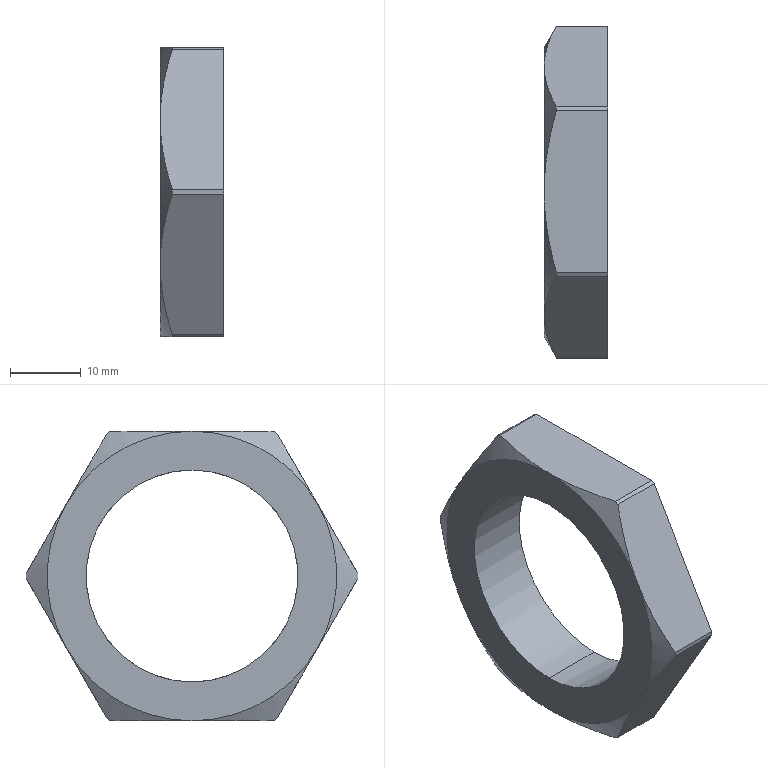Component | SolidWorks | MAL40_M30x2_Nut-1 | 1 solid | 22 faces | box 9 x 47 x 41 mm | volume 6663 mm3 | cylinder 8 | plane 8 | cone 6 | commonest cylinder face diameters 47 x6 30 x2
build123d program:
from build123d import *

# Parameters (mm, degrees)
SKETCH2_W                         = 82
SKETCH2_H                         = 82
EXTRUDE1_DEPTH                    = 18
THREADMAJORDIABORE_M30_DEPTH      = 33.458
THREADMAJORDIABORE_M30_DEPTH_BACK = 33.458
SKETCH4_R                         = 15


with BuildPart() as part:
    # Sketch1 → Revolve1 (revolve)
    with BuildSketch(Plane.XY, mode=Mode.PRIVATE) as revolve1_sk:
        Polygon((0, 0), (0, 20.5), (1.732, 23.5), (9, 23.5), (9, 0), align=None)
    revolve(revolve1_sk.sketch.rotate(Axis((9, 0, 0), (-1, 0, 0)), 270), axis=Axis((9, 0, 0), (-1, 0, 0)))

    # Sketch2 → Extrude1 (cut)
    with BuildSketch(Plane(origin=(0, 0, 0), x_dir=(0, 0, -1), z_dir=(1, 0, 0))):
        Rectangle(SKETCH2_W, SKETCH2_H)
        Polygon((-20.5, 11.836), (-20.5, -11.836), (0, -23.671), (20.5, -11.836), (20.5, 11.836), (0, 23.671), align=None, mode=Mode.SUBTRACT)
    extrude(amount=EXTRUDE1_DEPTH, mode=Mode.SUBTRACT)

    # Sketch3 → Cut-Revolve1 (revolve, cut)
    with BuildSketch(Plane.XY, mode=Mode.PRIVATE) as cut_revolve1_sk:
        Polygon((0, 0), (0, 15), (1.083, 13.918), (7.918, 13.918), (9, 15), (9, 0), align=None)
    revolve(cut_revolve1_sk.sketch.rotate(Axis((9, 0, 0), (-1, 0, 0)), 270), axis=Axis((9, 0, 0), (-1, 0, 0)), mode=Mode.SUBTRACT)

    # Sketch4 → ThreadMajorDiaBore_M30 (cut, two sides: drawn at the far end of the back side and taken through both)
    with BuildSketch(Plane(origin=(0, 0, 0), x_dir=(0, 0, -1), z_dir=(1, 0, 0)).offset(-THREADMAJORDIABORE_M30_DEPTH_BACK)):
        Circle(SKETCH4_R)
    extrude(amount=THREADMAJORDIABORE_M30_DEPTH + THREADMAJORDIABORE_M30_DEPTH_BACK, mode=Mode.SUBTRACT)


solid = part.part

# Placed as in the assembly
solid = solid.moved(Location((-14, 0, 0), (0, 0, 0)))
STEP:
#1=COLOUR_RGB('',0.7922,0.8196,0.9333);
#2=FILL_AREA_STYLE_COLOUR('',#1);
#3=FILL_AREA_STYLE('',(#2));
#4=SURFACE_STYLE_FILL_AREA(#3);
#5=SURFACE_SIDE_STYLE('',(#4));
#6=SURFACE_STYLE_USAGE(.BOTH.,#5);
#7=PRESENTATION_STYLE_ASSIGNMENT((#6));
#8=CARTESIAN_POINT('',(-0.5512,0.,0.5906));
#9=VERTEX_POINT('',#8);
#10=CARTESIAN_POINT('',(-0.5512,0.,-0.5906));
#11=VERTEX_POINT('',#10);
#12=CARTESIAN_POINT('',(-0.5512,0.,0.5906));
#13=CARTESIAN_POINT('',(-0.5512,-0.03877,0.5906));
#14=CARTESIAN_POINT('',(-0.5512,-0.07719,0.5868));
#15=CARTESIAN_POINT('',(-0.5512,-0.1532,0.5716));
#16=CARTESIAN_POINT('',(-0.5512,-0.1902,0.5604));
#17=CARTESIAN_POINT('',(-0.5512,-0.2618,0.5308));
#18=CARTESIAN_POINT('',(-0.5512,-0.2959,0.5126));
#19=CARTESIAN_POINT('',(-0.5512,-0.3603,0.4695));
#20=CARTESIAN_POINT('',(-0.5512,-0.3902,0.445));
#21=CARTESIAN_POINT('',(-0.5512,-0.445,0.3902));
#22=CARTESIAN_POINT('',(-0.5512,-0.4695,0.3603));
#23=CARTESIAN_POINT('',(-0.5512,-0.5126,0.2959));
#24=CARTESIAN_POINT('',(-0.5512,-0.5308,0.2618));
#25=CARTESIAN_POINT('',(-0.5512,-0.5604,0.1902));
#26=CARTESIAN_POINT('',(-0.5512,-0.5716,0.1532));
#27=CARTESIAN_POINT('',(-0.5512,-0.5868,0.07719));
#28=CARTESIAN_POINT('',(-0.5512,-0.5905,0.03876));
#29=CARTESIAN_POINT('',(-0.5512,-0.5906,-0.03876));
#30=CARTESIAN_POINT('',(-0.5512,-0.5868,-0.07719));
#31=CARTESIAN_POINT('',(-0.5512,-0.5716,-0.1532));
#32=CARTESIAN_POINT('',(-0.5512,-0.5604,-0.1902));
#33=CARTESIAN_POINT('',(-0.5512,-0.5308,-0.2618));
#34=CARTESIAN_POINT('',(-0.5512,-0.5126,-0.2959));
#35=CARTESIAN_POINT('',(-0.5512,-0.4695,-0.3603));
#36=CARTESIAN_POINT('',(-0.5512,-0.445,-0.3902));
#37=CARTESIAN_POINT('',(-0.5512,-0.3902,-0.445));
#38=CARTESIAN_POINT('',(-0.5512,-0.3603,-0.4695));
#39=CARTESIAN_POINT('',(-0.5512,-0.2959,-0.5126));
#40=CARTESIAN_POINT('',(-0.5512,-0.2618,-0.5308));
#41=CARTESIAN_POINT('',(-0.5512,-0.1902,-0.5604));
#42=CARTESIAN_POINT('',(-0.5512,-0.1532,-0.5716));
#43=CARTESIAN_POINT('',(-0.5512,-0.07719,-0.5868));
#44=CARTESIAN_POINT('',(-0.5512,-0.03876,-0.5905));
#45=CARTESIAN_POINT('',(-0.5512,0.,-0.5906));
#46=B_SPLINE_CURVE_WITH_KNOTS('',3,(#12,#13,#14,#15,#16,#17,#18,#19,#20,#21,#22,#23,#24,#25,#26,#27,#28,#29,#30,#31,#32,#33,#34,#35,#36,#37,#38,#39,#40,#41,#42,#43,#44,#45),.UNSPECIFIED.,.F.,.F.,(4,2,2,2,2,2,2,2,2,2,2,2,2,2,2,2,4),(0.,0.03125,0.0625,0.09375,0.125,0.1563,0.1875,0.2188,0.25,0.2813,0.3125,0.3438,0.375,0.4063,0.4375,0.4688,0.5),.UNSPECIFIED.);
#47=EDGE_CURVE('',#9,#11,#46,.T.);
#48=ORIENTED_EDGE('',*,*,#47,.F.);
#49=CARTESIAN_POINT('',(-0.1969,0.,0.5906));
#50=VERTEX_POINT('',#49);
#51=CARTESIAN_POINT('',(-0.5512,0.,0.5906));
#52=DIRECTION('',(1.,0.,0.));
#53=VECTOR('',#52,39.37);
#54=LINE('',#51,#53);
#55=EDGE_CURVE('',#9,#50,#54,.T.);
#56=ORIENTED_EDGE('',*,*,#55,.T.);
#57=CARTESIAN_POINT('',(-0.1969,0.,-0.5906));
#58=VERTEX_POINT('',#57);
#59=CARTESIAN_POINT('',(-0.1969,0.,0.));
#60=DIRECTION('',(1.,0.,0.));
#61=DIRECTION('',(0.,0.,-1.));
#62=AXIS2_PLACEMENT_3D('',#59,#60,#61);
#63=CIRCLE('',#62,0.5906);
#64=EDGE_CURVE('',#50,#58,#63,.T.);
#65=ORIENTED_EDGE('',*,*,#64,.T.);
#66=CARTESIAN_POINT('',(-0.5512,0.,-0.5906));
#67=DIRECTION('',(1.,0.,0.));
#68=VECTOR('',#67,39.37);
#69=LINE('',#66,#68);
#70=EDGE_CURVE('',#11,#58,#69,.T.);
#71=ORIENTED_EDGE('',*,*,#70,.F.);
#72=EDGE_LOOP('',(#48,#56,#65,#71));
#73=FACE_OUTER_BOUND('',#72,.T.);
#74=CARTESIAN_POINT('',(-0.5512,0.,0.));
#75=DIRECTION('',(1.,0.,0.));
#76=DIRECTION('',(0.,0.,-1.));
#77=AXIS2_PLACEMENT_3D('',#74,#75,#76);
#78=CYLINDRICAL_SURFACE('',#77,0.5906);
#79=ADVANCED_FACE('',(#73),#78,.F.);
#80=CARTESIAN_POINT('',(-0.5512,0.,0.8071));
#81=VERTEX_POINT('',#80);
#82=CARTESIAN_POINT('',(-0.5512,0.699,0.4035));
#83=VERTEX_POINT('',#82);
#84=CARTESIAN_POINT('',(-0.5512,0.,0.));
#85=DIRECTION('',(-1.,0.,0.));
#86=DIRECTION('',(0.,0.,1.));
#87=AXIS2_PLACEMENT_3D('',#84,#85,#86);
#88=CIRCLE('',#87,0.8071);
#89=EDGE_CURVE('',#81,#83,#88,.T.);
#90=ORIENTED_EDGE('',*,*,#89,.T.);
#91=CARTESIAN_POINT('',(-0.5512,0.699,-0.4035));
#92=VERTEX_POINT('',#91);
#93=CARTESIAN_POINT('',(-0.5512,0.,0.));
#94=DIRECTION('',(-1.,0.,0.));
#95=DIRECTION('',(0.,0.,1.));
#96=AXIS2_PLACEMENT_3D('',#93,#94,#95);
#97=CIRCLE('',#96,0.8071);
#98=EDGE_CURVE('',#83,#92,#97,.T.);
#99=ORIENTED_EDGE('',*,*,#98,.T.);
#100=CARTESIAN_POINT('',(-0.5512,0.,-0.8071));
#101=VERTEX_POINT('',#100);
#102=CARTESIAN_POINT('',(-0.5512,0.,0.));
#103=DIRECTION('',(-1.,0.,0.));
#104=DIRECTION('',(0.,0.,1.));
#105=AXIS2_PLACEMENT_3D('',#102,#103,#104);
#106=CIRCLE('',#105,0.8071);
#107=EDGE_CURVE('',#92,#101,#106,.T.);
#108=ORIENTED_EDGE('',*,*,#107,.T.);
#109=CARTESIAN_POINT('',(-0.5512,-0.699,-0.4035));
#110=VERTEX_POINT('',#109);
#111=CARTESIAN_POINT('',(-0.5512,0.,0.));
#112=DIRECTION('',(-1.,0.,0.));
#113=DIRECTION('',(0.,0.,1.));
#114=AXIS2_PLACEMENT_3D('',#111,#112,#113);
#115=CIRCLE('',#114,0.8071);
#116=EDGE_CURVE('',#101,#110,#115,.T.);
#117=ORIENTED_EDGE('',*,*,#116,.T.);
#118=CARTESIAN_POINT('',(-0.5512,-0.699,0.4035));
#119=VERTEX_POINT('',#118);
#120=CARTESIAN_POINT('',(-0.5512,0.,0.));
#121=DIRECTION('',(-1.,0.,0.));
#122=DIRECTION('',(0.,0.,1.));
#123=AXIS2_PLACEMENT_3D('',#120,#121,#122);
#124=CIRCLE('',#123,0.8071);
#125=EDGE_CURVE('',#110,#119,#124,.T.);
#126=ORIENTED_EDGE('',*,*,#125,.T.);
#127=CARTESIAN_POINT('',(-0.5512,0.,0.));
#128=DIRECTION('',(-1.,0.,0.));
#129=DIRECTION('',(0.,0.,1.));
#130=AXIS2_PLACEMENT_3D('',#127,#128,#129);
#131=CIRCLE('',#130,0.8071);
#132=EDGE_CURVE('',#119,#81,#131,.T.);
#133=ORIENTED_EDGE('',*,*,#132,.T.);
#134=EDGE_LOOP('',(#90,#99,#108,#117,#126,#133));
#135=FACE_OUTER_BOUND('',#134,.T.);
#136=CARTESIAN_POINT('',(-0.5512,0.,-0.5906));
#137=CARTESIAN_POINT('',(-0.5512,0.03876,-0.5906));
#138=CARTESIAN_POINT('',(-0.5512,0.07719,-0.5868));
#139=CARTESIAN_POINT('',(-0.5512,0.1532,-0.5716));
#140=CARTESIAN_POINT('',(-0.5512,0.1902,-0.5604));
#141=CARTESIAN_POINT('',(-0.5512,0.2618,-0.5308));
#142=CARTESIAN_POINT('',(-0.5512,0.2959,-0.5126));
#143=CARTESIAN_POINT('',(-0.5512,0.3603,-0.4695));
#144=CARTESIAN_POINT('',(-0.5512,0.3902,-0.445));
#145=CARTESIAN_POINT('',(-0.5512,0.445,-0.3902));
#146=CARTESIAN_POINT('',(-0.5512,0.4695,-0.3603));
#147=CARTESIAN_POINT('',(-0.5512,0.5126,-0.2959));
#148=CARTESIAN_POINT('',(-0.5512,0.5308,-0.2618));
#149=CARTESIAN_POINT('',(-0.5512,0.5604,-0.1902));
#150=CARTESIAN_POINT('',(-0.5512,0.5716,-0.1532));
#151=CARTESIAN_POINT('',(-0.5512,0.5868,-0.07719));
#152=CARTESIAN_POINT('',(-0.5512,0.5905,-0.03876));
#153=CARTESIAN_POINT('',(-0.5512,0.5906,0.03876));
#154=CARTESIAN_POINT('',(-0.5512,0.5868,0.07719));
#155=CARTESIAN_POINT('',(-0.5512,0.5716,0.1532));
#156=CARTESIAN_POINT('',(-0.5512,0.5604,0.1902));
#157=CARTESIAN_POINT('',(-0.5512,0.5308,0.2618));
#158=CARTESIAN_POINT('',(-0.5512,0.5126,0.2959));
#159=CARTESIAN_POINT('',(-0.5512,0.4695,0.3603));
#160=CARTESIAN_POINT('',(-0.5512,0.445,0.3902));
#161=CARTESIAN_POINT('',(-0.5512,0.3902,0.445));
#162=CARTESIAN_POINT('',(-0.5512,0.3603,0.4695));
#163=CARTESIAN_POINT('',(-0.5512,0.2959,0.5126));
#164=CARTESIAN_POINT('',(-0.5512,0.2618,0.5308));
#165=CARTESIAN_POINT('',(-0.5512,0.1902,0.5604));
#166=CARTESIAN_POINT('',(-0.5512,0.1532,0.5716));
#167=CARTESIAN_POINT('',(-0.5512,0.07719,0.5868));
#168=CARTESIAN_POINT('',(-0.5512,0.03878,0.5906));
#169=CARTESIAN_POINT('',(-0.5512,0.,0.5906));
#170=B_SPLINE_CURVE_WITH_KNOTS('',3,(#136,#137,#138,#139,#140,#141,#142,#143,#144,#145,#146,#147,#148,#149,#150,#151,#152,#153,#154,#155,#156,#157,#158,#159,#160,#161,#162,#163,#164,#165,#166,#167,#168,#169),.UNSPECIFIED.,.F.,.F.,(4,2,2,2,2,2,2,2,2,2,2,2,2,2,2,2,4),(0.5,0.5312,0.5625,0.5938,0.625,0.6562,0.6875,0.7188,0.75,0.7812,0.8125,0.8438,0.875,0.9062,0.9375,0.9688,1.),.UNSPECIFIED.);
#171=EDGE_CURVE('',#11,#9,#170,.T.);
#172=ORIENTED_EDGE('',*,*,#171,.T.);
#173=ORIENTED_EDGE('',*,*,#47,.T.);
#174=EDGE_LOOP('',(#172,#173));
#175=FACE_BOUND('',#174,.T.);
#176=CARTESIAN_POINT('',(-0.5512,0.,0.));
#177=DIRECTION('',(1.,0.,0.));
#178=DIRECTION('',(0.,0.,-1.));
#179=AXIS2_PLACEMENT_3D('',#176,#177,#178);
#180=PLANE('',#179);
#181=ADVANCED_FACE('',(#135,#175),#180,.F.);
#182=CARTESIAN_POINT('',(-0.1969,0.9251,0.01182));
#183=VERTEX_POINT('',#182);
#184=CARTESIAN_POINT('',(-0.1969,0.9251,-0.01182));
#185=VERTEX_POINT('',#184);
#186=CARTESIAN_POINT('',(-0.1969,0.,0.));
#187=DIRECTION('',(-1.,0.,0.));
#188=DIRECTION('',(0.,0.,1.));
#189=AXIS2_PLACEMENT_3D('',#186,#187,#188);
#190=CIRCLE('',#189,0.9252);
#191=EDGE_CURVE('',#183,#185,#190,.T.);
#192=ORIENTED_EDGE('',*,*,#191,.F.);
#193=CARTESIAN_POINT('',(-0.1969,0.4728,0.7953));
#194=VERTEX_POINT('',#193);
#195=CARTESIAN_POINT('',(-0.1969,0.9303,0.002921));
#196=DIRECTION('',(0.,-0.5,0.866));
#197=VECTOR('',#196,39.37);
#198=LINE('',#195,#197);
#199=EDGE_CURVE('',#183,#194,#198,.T.);
#200=ORIENTED_EDGE('',*,*,#199,.T.);
#201=CARTESIAN_POINT('',(-0.1969,0.4523,0.8071));
#202=VERTEX_POINT('',#201);
#203=CARTESIAN_POINT('',(-0.1969,0.,0.));
#204=DIRECTION('',(-1.,0.,0.));
#205=DIRECTION('',(0.,0.,1.));
#206=AXIS2_PLACEMENT_3D('',#203,#204,#205);
#207=CIRCLE('',#206,0.9252);
#208=EDGE_CURVE('',#202,#194,#207,.T.);
#209=ORIENTED_EDGE('',*,*,#208,.F.);
#210=CARTESIAN_POINT('',(-0.1969,-0.4523,0.8071));
#211=VERTEX_POINT('',#210);
#212=CARTESIAN_POINT('',(-0.1969,0.9252,0.8071));
#213=DIRECTION('',(0.,-1.,0.));
#214=VECTOR('',#213,39.37);
#215=LINE('',#212,#214);
#216=EDGE_CURVE('',#202,#211,#215,.T.);
#217=ORIENTED_EDGE('',*,*,#216,.T.);
#218=CARTESIAN_POINT('',(-0.1969,-0.4728,0.7953));
#219=VERTEX_POINT('',#218);
#220=CARTESIAN_POINT('',(-0.1969,0.,0.));
#221=DIRECTION('',(-1.,0.,0.));
#222=DIRECTION('',(0.,0.,1.));
#223=AXIS2_PLACEMENT_3D('',#220,#221,#222);
#224=CIRCLE('',#223,0.9252);
#225=EDGE_CURVE('',#219,#211,#224,.T.);
#226=ORIENTED_EDGE('',*,*,#225,.F.);
#227=CARTESIAN_POINT('',(-0.1969,-0.9251,0.01182));
#228=VERTEX_POINT('',#227);
#229=CARTESIAN_POINT('',(-0.1969,-0.4677,0.8042));
#230=DIRECTION('',(0.,-0.5,-0.866));
#231=VECTOR('',#230,39.37);
#232=LINE('',#229,#231);
#233=EDGE_CURVE('',#219,#228,#232,.T.);
#234=ORIENTED_EDGE('',*,*,#233,.T.);
#235=CARTESIAN_POINT('',(-0.1969,-0.9251,-0.01182));
#236=VERTEX_POINT('',#235);
#237=CARTESIAN_POINT('',(-0.1969,0.,0.));
#238=DIRECTION('',(-1.,0.,0.));
#239=DIRECTION('',(0.,0.,1.));
#240=AXIS2_PLACEMENT_3D('',#237,#238,#239);
#241=CIRCLE('',#240,0.9252);
#242=EDGE_CURVE('',#236,#228,#241,.T.);
#243=ORIENTED_EDGE('',*,*,#242,.F.);
#244=CARTESIAN_POINT('',(-0.1969,-0.4728,-0.7953));
#245=VERTEX_POINT('',#244);
#246=CARTESIAN_POINT('',(-0.1969,-0.4677,-0.8042));
#247=DIRECTION('',(0.,0.5,-0.866));
#248=VECTOR('',#247,39.37);
#249=LINE('',#246,#248);
#250=EDGE_CURVE('',#236,#245,#249,.T.);
#251=ORIENTED_EDGE('',*,*,#250,.T.);
#252=CARTESIAN_POINT('',(-0.1969,-0.4523,-0.8071));
#253=VERTEX_POINT('',#252);
#254=CARTESIAN_POINT('',(-0.1969,0.,0.));
#255=DIRECTION('',(-1.,0.,0.));
#256=DIRECTION('',(0.,0.,1.));
#257=AXIS2_PLACEMENT_3D('',#254,#255,#256);
#258=CIRCLE('',#257,0.9252);
#259=EDGE_CURVE('',#253,#245,#258,.T.);
#260=ORIENTED_EDGE('',*,*,#259,.F.);
#261=CARTESIAN_POINT('',(-0.1969,0.4523,-0.8071));
#262=VERTEX_POINT('',#261);
#263=CARTESIAN_POINT('',(-0.1969,0.9252,-0.8071));
#264=DIRECTION('',(0.,1.,0.));
#265=VECTOR('',#264,39.37);
#266=LINE('',#263,#265);
#267=EDGE_CURVE('',#253,#262,#266,.T.);
#268=ORIENTED_EDGE('',*,*,#267,.T.);
#269=CARTESIAN_POINT('',(-0.1969,0.4728,-0.7953));
#270=VERTEX_POINT('',#269);
#271=CARTESIAN_POINT('',(-0.1969,0.,0.));
#272=DIRECTION('',(-1.,0.,0.));
#273=DIRECTION('',(0.,0.,1.));
#274=AXIS2_PLACEMENT_3D('',#271,#272,#273);
#275=CIRCLE('',#274,0.9252);
#276=EDGE_CURVE('',#270,#262,#275,.T.);
#277=ORIENTED_EDGE('',*,*,#276,.F.);
#278=CARTESIAN_POINT('',(-0.1969,0.9303,-0.002921));
#279=DIRECTION('',(0.,0.5,0.866));
#280=VECTOR('',#279,39.37);
#281=LINE('',#278,#280);
#282=EDGE_CURVE('',#270,#185,#281,.T.);
#283=ORIENTED_EDGE('',*,*,#282,.T.);
#284=EDGE_LOOP('',(#192,#200,#209,#217,#226,#234,#243,#251,#260,#268,#277,#283));
#285=FACE_OUTER_BOUND('',#284,.T.);
#286=CARTESIAN_POINT('',(-0.1969,0.,0.));
#287=DIRECTION('',(1.,0.,0.));
#288=DIRECTION('',(0.,0.,-1.));
#289=AXIS2_PLACEMENT_3D('',#286,#287,#288);
#290=CIRCLE('',#289,0.5906);
#291=EDGE_CURVE('',#58,#50,#290,.T.);
#292=ORIENTED_EDGE('',*,*,#291,.F.);
#293=ORIENTED_EDGE('',*,*,#64,.F.);
#294=EDGE_LOOP('',(#292,#293));
#295=FACE_BOUND('',#294,.T.);
#296=CARTESIAN_POINT('',(-0.1969,0.9252,0.));
#297=DIRECTION('',(-1.,0.,0.));
#298=DIRECTION('',(0.,0.,1.));
#299=AXIS2_PLACEMENT_3D('',#296,#297,#298);
#300=PLANE('',#299);
#301=ADVANCED_FACE('',(#285,#295),#300,.F.);
#302=CARTESIAN_POINT('',(-0.483,0.4523,0.8071));
#303=VERTEX_POINT('',#302);
#304=CARTESIAN_POINT('',(-0.483,0.4728,0.7953));
#305=VERTEX_POINT('',#304);
#306=CARTESIAN_POINT('',(-0.483,0.,0.));
#307=DIRECTION('',(-1.,0.,0.));
#308=DIRECTION('',(0.,0.,1.));
#309=AXIS2_PLACEMENT_3D('',#306,#307,#308);
#310=CIRCLE('',#309,0.9252);
#311=EDGE_CURVE('',#303,#305,#310,.T.);
#312=ORIENTED_EDGE('',*,*,#311,.T.);
#313=CARTESIAN_POINT('',(-0.483,0.4728,0.7953));
#314=CARTESIAN_POINT('',(-0.5039,0.5098,0.7311));
#315=CARTESIAN_POINT('',(-0.5211,0.5471,0.6665));
#316=CARTESIAN_POINT('',(-0.5447,0.6225,0.536));
#317=CARTESIAN_POINT('',(-0.5512,0.6605,0.4702));
#318=CARTESIAN_POINT('',(-0.5512,0.699,0.4035));
#319=B_SPLINE_CURVE_WITH_KNOTS('',3,(#313,#314,#315,#316,#317,#318),.UNSPECIFIED.,.F.,.F.,(4,2,4),(0.00000073,0.00581,0.01162),.UNSPECIFIED.);
#320=EDGE_CURVE('',#305,#83,#319,.T.);
#321=ORIENTED_EDGE('',*,*,#320,.T.);
#322=ORIENTED_EDGE('',*,*,#89,.F.);
#323=CARTESIAN_POINT('',(-0.5512,0.,0.8071));
#324=CARTESIAN_POINT('',(-0.5512,0.03821,0.8071));
#325=CARTESIAN_POINT('',(-0.5496,0.07653,0.8071));
#326=CARTESIAN_POINT('',(-0.5433,0.1534,0.8071));
#327=CARTESIAN_POINT('',(-0.5387,0.1916,0.8071));
#328=CARTESIAN_POINT('',(-0.5208,0.305,0.8071));
#329=CARTESIAN_POINT('',(-0.5036,0.3791,0.8071));
#330=CARTESIAN_POINT('',(-0.483,0.4523,0.8071));
#331=B_SPLINE_CURVE_WITH_KNOTS('',3,(#323,#324,#325,#326,#327,#328,#329,#330),.UNSPECIFIED.,.F.,.F.,(4,2,2,4),(0.03307,0.03598,0.03888,0.04469),.UNSPECIFIED.);
#332=EDGE_CURVE('',#81,#303,#331,.T.);
#333=ORIENTED_EDGE('',*,*,#332,.T.);
#334=EDGE_LOOP('',(#312,#321,#322,#333));
#335=FACE_OUTER_BOUND('',#334,.T.);
#336=CARTESIAN_POINT('',(-0.483,0.,0.));
#337=DIRECTION('',(1.,0.,0.));
#338=DIRECTION('',(0.,0.,-1.));
#339=AXIS2_PLACEMENT_3D('',#336,#337,#338);
#340=CONICAL_SURFACE('',#339,0.9252,1.047);
#341=ADVANCED_FACE('',(#335),#340,.T.);
#342=CARTESIAN_POINT('',(-0.483,-0.4728,0.7953));
#343=VERTEX_POINT('',#342);
#344=CARTESIAN_POINT('',(-0.483,-0.4523,0.8071));
#345=VERTEX_POINT('',#344);
#346=CARTESIAN_POINT('',(-0.483,0.,0.));
#347=DIRECTION('',(-1.,0.,0.));
#348=DIRECTION('',(0.,0.,1.));
#349=AXIS2_PLACEMENT_3D('',#346,#347,#348);
#350=CIRCLE('',#349,0.9252);
#351=EDGE_CURVE('',#343,#345,#350,.T.);
#352=ORIENTED_EDGE('',*,*,#351,.T.);
#353=CARTESIAN_POINT('',(-0.483,-0.4523,0.8071));
#354=CARTESIAN_POINT('',(-0.4934,-0.4155,0.8071));
#355=CARTESIAN_POINT('',(-0.5029,-0.3783,0.8071));
#356=CARTESIAN_POINT('',(-0.5198,-0.3032,0.8071));
#357=CARTESIAN_POINT('',(-0.5271,-0.2655,0.8071));
#358=CARTESIAN_POINT('',(-0.5448,-0.1523,0.8071));
#359=CARTESIAN_POINT('',(-0.5512,-0.07638,0.8071));
#360=CARTESIAN_POINT('',(-0.5512,0.,0.8071));
#361=B_SPLINE_CURVE_WITH_KNOTS('',3,(#353,#354,#355,#356,#357,#358,#359,#360),.UNSPECIFIED.,.F.,.F.,(4,2,2,4),(0.02146,0.02436,0.02727,0.03307),.UNSPECIFIED.);
#362=EDGE_CURVE('',#345,#81,#361,.T.);
#363=ORIENTED_EDGE('',*,*,#362,.T.);
#364=ORIENTED_EDGE('',*,*,#132,.F.);
#365=CARTESIAN_POINT('',(-0.5512,-0.699,0.4035));
#366=CARTESIAN_POINT('',(-0.5512,-0.6798,0.4367));
#367=CARTESIAN_POINT('',(-0.5496,-0.6605,0.4701));
#368=CARTESIAN_POINT('',(-0.5434,-0.6224,0.5361));
#369=CARTESIAN_POINT('',(-0.5388,-0.6035,0.5689));
#370=CARTESIAN_POINT('',(-0.521,-0.547,0.6668));
#371=CARTESIAN_POINT('',(-0.5038,-0.5097,0.7313));
#372=CARTESIAN_POINT('',(-0.483,-0.4728,0.7953));
#373=B_SPLINE_CURVE_WITH_KNOTS('',3,(#365,#366,#367,#368,#369,#370,#371,#372),.UNSPECIFIED.,.F.,.F.,(4,2,2,4),(0.01162,0.01451,0.0174,0.02318),.UNSPECIFIED.);
#374=EDGE_CURVE('',#119,#343,#373,.T.);
#375=ORIENTED_EDGE('',*,*,#374,.T.);
#376=EDGE_LOOP('',(#352,#363,#364,#375));
#377=FACE_OUTER_BOUND('',#376,.T.);
#378=CARTESIAN_POINT('',(-0.483,0.,0.));
#379=DIRECTION('',(1.,0.,0.));
#380=DIRECTION('',(0.,0.,-1.));
#381=AXIS2_PLACEMENT_3D('',#378,#379,#380);
#382=CONICAL_SURFACE('',#381,0.9252,1.047);
#383=ADVANCED_FACE('',(#377),#382,.T.);
#384=CARTESIAN_POINT('',(-0.483,-0.9251,-0.01182));
#385=VERTEX_POINT('',#384);
#386=CARTESIAN_POINT('',(-0.483,-0.9251,0.01182));
#387=VERTEX_POINT('',#386);
#388=CARTESIAN_POINT('',(-0.483,0.,0.));
#389=DIRECTION('',(-1.,0.,0.));
#390=DIRECTION('',(0.,0.,1.));
#391=AXIS2_PLACEMENT_3D('',#388,#389,#390);
#392=CIRCLE('',#391,0.9252);
#393=EDGE_CURVE('',#385,#387,#392,.T.);
#394=ORIENTED_EDGE('',*,*,#393,.T.);
#395=CARTESIAN_POINT('',(-0.483,-0.9251,0.01182));
#396=CARTESIAN_POINT('',(-0.5039,-0.8881,0.07598));
#397=CARTESIAN_POINT('',(-0.5211,-0.8508,0.1406));
#398=CARTESIAN_POINT('',(-0.5447,-0.7755,0.271));
#399=CARTESIAN_POINT('',(-0.5512,-0.7374,0.3369));
#400=CARTESIAN_POINT('',(-0.5512,-0.699,0.4035));
#401=B_SPLINE_CURVE_WITH_KNOTS('',3,(#395,#396,#397,#398,#399,#400),.UNSPECIFIED.,.F.,.F.,(4,2,4),(0.00000073,0.00581,0.01162),.UNSPECIFIED.);
#402=EDGE_CURVE('',#387,#119,#401,.T.);
#403=ORIENTED_EDGE('',*,*,#402,.T.);
#404=ORIENTED_EDGE('',*,*,#125,.F.);
#405=CARTESIAN_POINT('',(-0.5512,-0.699,-0.4035));
#406=CARTESIAN_POINT('',(-0.5512,-0.7181,-0.3704));
#407=CARTESIAN_POINT('',(-0.5496,-0.7374,-0.337));
#408=CARTESIAN_POINT('',(-0.5434,-0.7755,-0.271));
#409=CARTESIAN_POINT('',(-0.5388,-0.7945,-0.2381));
#410=CARTESIAN_POINT('',(-0.521,-0.851,-0.1403));
#411=CARTESIAN_POINT('',(-0.5038,-0.8882,-0.07578));
#412=CARTESIAN_POINT('',(-0.483,-0.9251,-0.01182));
#413=B_SPLINE_CURVE_WITH_KNOTS('',3,(#405,#406,#407,#408,#409,#410,#411,#412),.UNSPECIFIED.,.F.,.F.,(4,2,2,4),(0.01162,0.01451,0.0174,0.02318),.UNSPECIFIED.);
#414=EDGE_CURVE('',#110,#385,#413,.T.);
#415=ORIENTED_EDGE('',*,*,#414,.T.);
#416=EDGE_LOOP('',(#394,#403,#404,#415));
#417=FACE_OUTER_BOUND('',#416,.T.);
#418=CARTESIAN_POINT('',(-0.483,0.,0.));
#419=DIRECTION('',(1.,0.,0.));
#420=DIRECTION('',(0.,0.,-1.));
#421=AXIS2_PLACEMENT_3D('',#418,#419,#420);
#422=CONICAL_SURFACE('',#421,0.9252,1.047);
#423=ADVANCED_FACE('',(#417),#422,.T.);
#424=CARTESIAN_POINT('',(-0.483,-0.4523,-0.8071));
#425=VERTEX_POINT('',#424);
#426=CARTESIAN_POINT('',(-0.483,-0.4728,-0.7953));
#427=VERTEX_POINT('',#426);
#428=CARTESIAN_POINT('',(-0.483,0.,0.));
#429=DIRECTION('',(-1.,0.,0.));
#430=DIRECTION('',(0.,0.,1.));
#431=AXIS2_PLACEMENT_3D('',#428,#429,#430);
#432=CIRCLE('',#431,0.9252);
#433=EDGE_CURVE('',#425,#427,#432,.T.);
#434=ORIENTED_EDGE('',*,*,#433,.T.);
#435=CARTESIAN_POINT('',(-0.483,-0.4728,-0.7953));
#436=CARTESIAN_POINT('',(-0.5039,-0.5098,-0.7311));
#437=CARTESIAN_POINT('',(-0.5211,-0.5471,-0.6665));
#438=CARTESIAN_POINT('',(-0.5447,-0.6225,-0.536));
#439=CARTESIAN_POINT('',(-0.5512,-0.6605,-0.4702));
#440=CARTESIAN_POINT('',(-0.5512,-0.699,-0.4035));
#441=B_SPLINE_CURVE_WITH_KNOTS('',3,(#435,#436,#437,#438,#439,#440),.UNSPECIFIED.,.F.,.F.,(4,2,4),(0.00000073,0.00581,0.01162),.UNSPECIFIED.);
#442=EDGE_CURVE('',#427,#110,#441,.T.);
#443=ORIENTED_EDGE('',*,*,#442,.T.);
#444=ORIENTED_EDGE('',*,*,#116,.F.);
#445=CARTESIAN_POINT('',(-0.5512,0.,-0.8071));
#446=CARTESIAN_POINT('',(-0.5512,-0.07638,-0.8071));
#447=CARTESIAN_POINT('',(-0.5448,-0.1523,-0.8071));
#448=CARTESIAN_POINT('',(-0.5271,-0.2655,-0.8071));
#449=CARTESIAN_POINT('',(-0.5198,-0.3032,-0.8071));
#450=CARTESIAN_POINT('',(-0.5029,-0.3783,-0.8071));
#451=CARTESIAN_POINT('',(-0.4934,-0.4155,-0.8071));
#452=CARTESIAN_POINT('',(-0.483,-0.4523,-0.8071));
#453=B_SPLINE_CURVE_WITH_KNOTS('',3,(#445,#446,#447,#448,#449,#450,#451,#452),.UNSPECIFIED.,.F.,.F.,(4,2,2,4),(0.02064,0.02643,0.02933,0.03223),.UNSPECIFIED.);
#454=EDGE_CURVE('',#101,#425,#453,.T.);
#455=ORIENTED_EDGE('',*,*,#454,.T.);
#456=EDGE_LOOP('',(#434,#443,#444,#455));
#457=FACE_OUTER_BOUND('',#456,.T.);
#458=CARTESIAN_POINT('',(-0.483,0.,0.));
#459=DIRECTION('',(1.,0.,0.));
#460=DIRECTION('',(0.,0.,-1.));
#461=AXIS2_PLACEMENT_3D('',#458,#459,#460);
#462=CONICAL_SURFACE('',#461,0.9252,1.047);
#463=ADVANCED_FACE('',(#457),#462,.T.);
#464=CARTESIAN_POINT('',(-0.483,0.4728,-0.7953));
#465=VERTEX_POINT('',#464);
#466=CARTESIAN_POINT('',(-0.483,0.4523,-0.8071));
#467=VERTEX_POINT('',#466);
#468=CARTESIAN_POINT('',(-0.483,0.,0.));
#469=DIRECTION('',(-1.,0.,0.));
#470=DIRECTION('',(0.,0.,1.));
#471=AXIS2_PLACEMENT_3D('',#468,#469,#470);
#472=CIRCLE('',#471,0.9252);
#473=EDGE_CURVE('',#465,#467,#472,.T.);
#474=ORIENTED_EDGE('',*,*,#473,.T.);
#475=CARTESIAN_POINT('',(-0.483,0.4523,-0.8071));
#476=CARTESIAN_POINT('',(-0.5036,0.3791,-0.8071));
#477=CARTESIAN_POINT('',(-0.5208,0.305,-0.8071));
#478=CARTESIAN_POINT('',(-0.5387,0.1916,-0.8071));
#479=CARTESIAN_POINT('',(-0.5433,0.1534,-0.8071));
#480=CARTESIAN_POINT('',(-0.5496,0.07653,-0.8071));
#481=CARTESIAN_POINT('',(-0.5512,0.03821,-0.8071));
#482=CARTESIAN_POINT('',(-0.5512,0.,-0.8071));
#483=B_SPLINE_CURVE_WITH_KNOTS('',3,(#475,#476,#477,#478,#479,#480,#481,#482),.UNSPECIFIED.,.F.,.F.,(4,2,2,4),(0.009053,0.01485,0.01774,0.02064),.UNSPECIFIED.);
#484=EDGE_CURVE('',#467,#101,#483,.T.);
#485=ORIENTED_EDGE('',*,*,#484,.T.);
#486=ORIENTED_EDGE('',*,*,#107,.F.);
#487=CARTESIAN_POINT('',(-0.5512,0.699,-0.4035));
#488=CARTESIAN_POINT('',(-0.5512,0.6798,-0.4367));
#489=CARTESIAN_POINT('',(-0.5496,0.6605,-0.4701));
#490=CARTESIAN_POINT('',(-0.5434,0.6224,-0.5361));
#491=CARTESIAN_POINT('',(-0.5388,0.6035,-0.5689));
#492=CARTESIAN_POINT('',(-0.521,0.547,-0.6668));
#493=CARTESIAN_POINT('',(-0.5038,0.5097,-0.7313));
#494=CARTESIAN_POINT('',(-0.483,0.4728,-0.7953));
#495=B_SPLINE_CURVE_WITH_KNOTS('',3,(#487,#488,#489,#490,#491,#492,#493,#494),.UNSPECIFIED.,.F.,.F.,(4,2,2,4),(0.01162,0.01451,0.0174,0.02318),.UNSPECIFIED.);
#496=EDGE_CURVE('',#92,#465,#495,.T.);
#497=ORIENTED_EDGE('',*,*,#496,.T.);
#498=EDGE_LOOP('',(#474,#485,#486,#497));
#499=FACE_OUTER_BOUND('',#498,.T.);
#500=CARTESIAN_POINT('',(-0.483,0.,0.));
#501=DIRECTION('',(1.,0.,0.));
#502=DIRECTION('',(0.,0.,-1.));
#503=AXIS2_PLACEMENT_3D('',#500,#501,#502);
#504=CONICAL_SURFACE('',#503,0.9252,1.047);
#505=ADVANCED_FACE('',(#499),#504,.T.);
#506=ORIENTED_EDGE('',*,*,#208,.T.);
#507=CARTESIAN_POINT('',(-0.1969,0.4728,0.7953));
#508=DIRECTION('',(-1.,0.,0.));
#509=VECTOR('',#508,39.37);
#510=LINE('',#507,#509);
#511=EDGE_CURVE('',#194,#305,#510,.T.);
#512=ORIENTED_EDGE('',*,*,#511,.T.);
#513=ORIENTED_EDGE('',*,*,#311,.F.);
#514=CARTESIAN_POINT('',(-0.1969,0.4523,0.8071));
#515=DIRECTION('',(1.,0.,0.));
#516=VECTOR('',#515,39.37);
#517=LINE('',#514,#516);
#518=EDGE_CURVE('',#303,#202,#517,.T.);
#519=ORIENTED_EDGE('',*,*,#518,.T.);
#520=EDGE_LOOP('',(#506,#512,#513,#519));
#521=FACE_OUTER_BOUND('',#520,.T.);
#522=CARTESIAN_POINT('',(-0.1969,0.,0.));
#523=DIRECTION('',(-1.,0.,0.));
#524=DIRECTION('',(0.,0.,1.));
#525=AXIS2_PLACEMENT_3D('',#522,#523,#524);
#526=CYLINDRICAL_SURFACE('',#525,0.9252);
#527=ADVANCED_FACE('',(#521),#526,.T.);
#528=ORIENTED_EDGE('',*,*,#225,.T.);
#529=CARTESIAN_POINT('',(-0.1969,-0.4523,0.8071));
#530=DIRECTION('',(-1.,0.,0.));
#531=VECTOR('',#530,39.37);
#532=LINE('',#529,#531);
#533=EDGE_CURVE('',#211,#345,#532,.T.);
#534=ORIENTED_EDGE('',*,*,#533,.T.);
#535=ORIENTED_EDGE('',*,*,#351,.F.);
#536=CARTESIAN_POINT('',(-0.1969,-0.4728,0.7953));
#537=DIRECTION('',(1.,0.,0.));
#538=VECTOR('',#537,39.37);
#539=LINE('',#536,#538);
#540=EDGE_CURVE('',#343,#219,#539,.T.);
#541=ORIENTED_EDGE('',*,*,#540,.T.);
#542=EDGE_LOOP('',(#528,#534,#535,#541));
#543=FACE_OUTER_BOUND('',#542,.T.);
#544=CARTESIAN_POINT('',(-0.1969,0.,0.));
#545=DIRECTION('',(-1.,0.,0.));
#546=DIRECTION('',(0.,0.,1.));
#547=AXIS2_PLACEMENT_3D('',#544,#545,#546);
#548=CYLINDRICAL_SURFACE('',#547,0.9252);
#549=ADVANCED_FACE('',(#543),#548,.T.);
#550=ORIENTED_EDGE('',*,*,#242,.T.);
#551=CARTESIAN_POINT('',(-0.1969,-0.9251,0.01182));
#552=DIRECTION('',(-1.,0.,0.));
#553=VECTOR('',#552,39.37);
#554=LINE('',#551,#553);
#555=EDGE_CURVE('',#228,#387,#554,.T.);
#556=ORIENTED_EDGE('',*,*,#555,.T.);
#557=ORIENTED_EDGE('',*,*,#393,.F.);
#558=CARTESIAN_POINT('',(-0.1969,-0.9251,-0.01182));
#559=DIRECTION('',(1.,0.,0.));
#560=VECTOR('',#559,39.37);
#561=LINE('',#558,#560);
#562=EDGE_CURVE('',#385,#236,#561,.T.);
#563=ORIENTED_EDGE('',*,*,#562,.T.);
#564=EDGE_LOOP('',(#550,#556,#557,#563));
#565=FACE_OUTER_BOUND('',#564,.T.);
#566=CARTESIAN_POINT('',(-0.1969,0.,0.));
#567=DIRECTION('',(-1.,0.,0.));
#568=DIRECTION('',(0.,0.,1.));
#569=AXIS2_PLACEMENT_3D('',#566,#567,#568);
#570=CYLINDRICAL_SURFACE('',#569,0.9252);
#571=ADVANCED_FACE('',(#565),#570,.T.);
#572=ORIENTED_EDGE('',*,*,#259,.T.);
#573=CARTESIAN_POINT('',(-0.1969,-0.4728,-0.7953));
#574=DIRECTION('',(-1.,0.,0.));
#575=VECTOR('',#574,39.37);
#576=LINE('',#573,#575);
#577=EDGE_CURVE('',#245,#427,#576,.T.);
#578=ORIENTED_EDGE('',*,*,#577,.T.);
#579=ORIENTED_EDGE('',*,*,#433,.F.);
#580=CARTESIAN_POINT('',(-0.1969,-0.4523,-0.8071));
#581=DIRECTION('',(1.,0.,0.));
#582=VECTOR('',#581,39.37);
#583=LINE('',#580,#582);
#584=EDGE_CURVE('',#425,#253,#583,.T.);
#585=ORIENTED_EDGE('',*,*,#584,.T.);
#586=EDGE_LOOP('',(#572,#578,#579,#585));
#587=FACE_OUTER_BOUND('',#586,.T.);
#588=CARTESIAN_POINT('',(-0.1969,0.,0.));
#589=DIRECTION('',(-1.,0.,0.));
#590=DIRECTION('',(0.,0.,1.));
#591=AXIS2_PLACEMENT_3D('',#588,#589,#590);
#592=CYLINDRICAL_SURFACE('',#591,0.9252);
#593=ADVANCED_FACE('',(#587),#592,.T.);
#594=ORIENTED_EDGE('',*,*,#276,.T.);
#595=CARTESIAN_POINT('',(-0.1969,0.4523,-0.8071));
#596=DIRECTION('',(-1.,0.,0.));
#597=VECTOR('',#596,39.37);
#598=LINE('',#595,#597);
#599=EDGE_CURVE('',#262,#467,#598,.T.);
#600=ORIENTED_EDGE('',*,*,#599,.T.);
#601=ORIENTED_EDGE('',*,*,#473,.F.);
#602=CARTESIAN_POINT('',(-0.1969,0.4728,-0.7953));
#603=DIRECTION('',(1.,0.,0.));
#604=VECTOR('',#603,39.37);
#605=LINE('',#602,#604);
#606=EDGE_CURVE('',#465,#270,#605,.T.);
#607=ORIENTED_EDGE('',*,*,#606,.T.);
#608=EDGE_LOOP('',(#594,#600,#601,#607));
#609=FACE_OUTER_BOUND('',#608,.T.);
#610=CARTESIAN_POINT('',(-0.1969,0.,0.));
#611=DIRECTION('',(-1.,0.,0.));
#612=DIRECTION('',(0.,0.,1.));
#613=AXIS2_PLACEMENT_3D('',#610,#611,#612);
#614=CYLINDRICAL_SURFACE('',#613,0.9252);
#615=ADVANCED_FACE('',(#609),#614,.T.);
#616=ORIENTED_EDGE('',*,*,#98,.F.);
#617=CARTESIAN_POINT('',(-0.483,0.9251,0.01182));
#618=VERTEX_POINT('',#617);
#619=CARTESIAN_POINT('',(-0.5512,0.699,0.4035));
#620=CARTESIAN_POINT('',(-0.5512,0.7181,0.3704));
#621=CARTESIAN_POINT('',(-0.5496,0.7374,0.337));
#622=CARTESIAN_POINT('',(-0.5434,0.7755,0.271));
#623=CARTESIAN_POINT('',(-0.5388,0.7945,0.2381));
#624=CARTESIAN_POINT('',(-0.521,0.851,0.1403));
#625=CARTESIAN_POINT('',(-0.5038,0.8882,0.07578));
#626=CARTESIAN_POINT('',(-0.483,0.9251,0.01182));
#627=B_SPLINE_CURVE_WITH_KNOTS('',3,(#619,#620,#621,#622,#623,#624,#625,#626),.UNSPECIFIED.,.F.,.F.,(4,2,2,4),(0.01162,0.01451,0.0174,0.02318),.UNSPECIFIED.);
#628=EDGE_CURVE('',#83,#618,#627,.T.);
#629=ORIENTED_EDGE('',*,*,#628,.T.);
#630=CARTESIAN_POINT('',(-0.483,0.9251,-0.01182));
#631=VERTEX_POINT('',#630);
#632=CARTESIAN_POINT('',(-0.483,0.,0.));
#633=DIRECTION('',(-1.,0.,0.));
#634=DIRECTION('',(0.,0.,1.));
#635=AXIS2_PLACEMENT_3D('',#632,#633,#634);
#636=CIRCLE('',#635,0.9252);
#637=EDGE_CURVE('',#618,#631,#636,.T.);
#638=ORIENTED_EDGE('',*,*,#637,.T.);
#639=CARTESIAN_POINT('',(-0.483,0.9251,-0.01182));
#640=CARTESIAN_POINT('',(-0.5039,0.8881,-0.07598));
#641=CARTESIAN_POINT('',(-0.5211,0.8508,-0.1406));
#642=CARTESIAN_POINT('',(-0.5447,0.7755,-0.271));
#643=CARTESIAN_POINT('',(-0.5512,0.7374,-0.3369));
#644=CARTESIAN_POINT('',(-0.5512,0.699,-0.4035));
#645=B_SPLINE_CURVE_WITH_KNOTS('',3,(#639,#640,#641,#642,#643,#644),.UNSPECIFIED.,.F.,.F.,(4,2,4),(0.00000073,0.00581,0.01162),.UNSPECIFIED.);
#646=EDGE_CURVE('',#631,#92,#645,.T.);
#647=ORIENTED_EDGE('',*,*,#646,.T.);
#648=EDGE_LOOP('',(#616,#629,#638,#647));
#649=FACE_OUTER_BOUND('',#648,.T.);
#650=CARTESIAN_POINT('',(-0.483,0.,0.));
#651=DIRECTION('',(1.,0.,0.));
#652=DIRECTION('',(0.,0.,-1.));
#653=AXIS2_PLACEMENT_3D('',#650,#651,#652);
#654=CONICAL_SURFACE('',#653,0.9252,1.047);
#655=ADVANCED_FACE('',(#649),#654,.T.);
#656=ORIENTED_EDGE('',*,*,#637,.F.);
#657=CARTESIAN_POINT('',(-0.1969,0.9251,0.01182));
#658=DIRECTION('',(1.,0.,0.));
#659=VECTOR('',#658,39.37);
#660=LINE('',#657,#659);
#661=EDGE_CURVE('',#618,#183,#660,.T.);
#662=ORIENTED_EDGE('',*,*,#661,.T.);
#663=ORIENTED_EDGE('',*,*,#191,.T.);
#664=CARTESIAN_POINT('',(-0.1969,0.9251,-0.01182));
#665=DIRECTION('',(-1.,0.,0.));
#666=VECTOR('',#665,39.37);
#667=LINE('',#664,#666);
#668=EDGE_CURVE('',#185,#631,#667,.T.);
#669=ORIENTED_EDGE('',*,*,#668,.T.);
#670=EDGE_LOOP('',(#656,#662,#663,#669));
#671=FACE_OUTER_BOUND('',#670,.T.);
#672=CARTESIAN_POINT('',(-0.1969,0.,0.));
#673=DIRECTION('',(-1.,0.,0.));
#674=DIRECTION('',(0.,0.,1.));
#675=AXIS2_PLACEMENT_3D('',#672,#673,#674);
#676=CYLINDRICAL_SURFACE('',#675,0.9252);
#677=ADVANCED_FACE('',(#671),#676,.T.);
#678=ORIENTED_EDGE('',*,*,#668,.F.);
#679=ORIENTED_EDGE('',*,*,#282,.F.);
#680=ORIENTED_EDGE('',*,*,#606,.F.);
#681=ORIENTED_EDGE('',*,*,#496,.F.);
#682=ORIENTED_EDGE('',*,*,#646,.F.);
#683=EDGE_LOOP('',(#678,#679,#680,#681,#682));
#684=FACE_OUTER_BOUND('',#683,.T.);
#685=CARTESIAN_POINT('',(0.1575,0.466,-0.8071));
#686=DIRECTION('',(0.,-0.866,0.5));
#687=DIRECTION('',(0.,-0.5,-0.866));
#688=AXIS2_PLACEMENT_3D('',#685,#686,#687);
#689=PLANE('',#688);
#690=ADVANCED_FACE('',(#684),#689,.F.);
#691=ORIENTED_EDGE('',*,*,#599,.F.);
#692=ORIENTED_EDGE('',*,*,#267,.F.);
#693=ORIENTED_EDGE('',*,*,#584,.F.);
#694=ORIENTED_EDGE('',*,*,#454,.F.);
#695=ORIENTED_EDGE('',*,*,#484,.F.);
#696=EDGE_LOOP('',(#691,#692,#693,#694,#695));
#697=FACE_OUTER_BOUND('',#696,.T.);
#698=CARTESIAN_POINT('',(0.1575,-0.466,-0.8071));
#699=DIRECTION('',(0.,0.,1.));
#700=DIRECTION('',(1.,0.,0.));
#701=AXIS2_PLACEMENT_3D('',#698,#699,#700);
#702=PLANE('',#701);
#703=ADVANCED_FACE('',(#697),#702,.F.);
#704=ORIENTED_EDGE('',*,*,#577,.F.);
#705=ORIENTED_EDGE('',*,*,#250,.F.);
#706=ORIENTED_EDGE('',*,*,#562,.F.);
#707=ORIENTED_EDGE('',*,*,#414,.F.);
#708=ORIENTED_EDGE('',*,*,#442,.F.);
#709=EDGE_LOOP('',(#704,#705,#706,#707,#708));
#710=FACE_OUTER_BOUND('',#709,.T.);
#711=CARTESIAN_POINT('',(0.1575,-0.9319,0.));
#712=DIRECTION('',(0.,0.866,0.5));
#713=DIRECTION('',(0.,-0.5,0.866));
#714=AXIS2_PLACEMENT_3D('',#711,#712,#713);
#715=PLANE('',#714);
#716=ADVANCED_FACE('',(#710),#715,.F.);
#717=ORIENTED_EDGE('',*,*,#555,.F.);
#718=ORIENTED_EDGE('',*,*,#233,.F.);
#719=ORIENTED_EDGE('',*,*,#540,.F.);
#720=ORIENTED_EDGE('',*,*,#374,.F.);
#721=ORIENTED_EDGE('',*,*,#402,.F.);
#722=EDGE_LOOP('',(#717,#718,#719,#720,#721));
#723=FACE_OUTER_BOUND('',#722,.T.);
#724=CARTESIAN_POINT('',(0.1575,-0.466,0.8071));
#725=DIRECTION('',(0.,0.866,-0.5));
#726=DIRECTION('',(0.,0.5,0.866));
#727=AXIS2_PLACEMENT_3D('',#724,#725,#726);
#728=PLANE('',#727);
#729=ADVANCED_FACE('',(#723),#728,.F.);
#730=ORIENTED_EDGE('',*,*,#533,.F.);
#731=ORIENTED_EDGE('',*,*,#216,.F.);
#732=ORIENTED_EDGE('',*,*,#518,.F.);
#733=ORIENTED_EDGE('',*,*,#332,.F.);
#734=ORIENTED_EDGE('',*,*,#362,.F.);
#735=EDGE_LOOP('',(#730,#731,#732,#733,#734));
#736=FACE_OUTER_BOUND('',#735,.T.);
#737=CARTESIAN_POINT('',(0.1575,0.466,0.8071));
#738=DIRECTION('',(0.,0.,-1.));
#739=DIRECTION('',(-1.,0.,0.));
#740=AXIS2_PLACEMENT_3D('',#737,#738,#739);
#741=PLANE('',#740);
#742=ADVANCED_FACE('',(#736),#741,.F.);
#743=ORIENTED_EDGE('',*,*,#511,.F.);
#744=ORIENTED_EDGE('',*,*,#199,.F.);
#745=ORIENTED_EDGE('',*,*,#661,.F.);
#746=ORIENTED_EDGE('',*,*,#628,.F.);
#747=ORIENTED_EDGE('',*,*,#320,.F.);
#748=EDGE_LOOP('',(#743,#744,#745,#746,#747));
#749=FACE_OUTER_BOUND('',#748,.T.);
#750=CARTESIAN_POINT('',(0.1575,0.9319,0.));
#751=DIRECTION('',(0.,-0.866,-0.5));
#752=DIRECTION('',(0.,0.5,-0.866));
#753=AXIS2_PLACEMENT_3D('',#750,#751,#752);
#754=PLANE('',#753);
#755=ADVANCED_FACE('',(#749),#754,.F.);
#756=ORIENTED_EDGE('',*,*,#55,.F.);
#757=ORIENTED_EDGE('',*,*,#171,.F.);
#758=ORIENTED_EDGE('',*,*,#70,.T.);
#759=ORIENTED_EDGE('',*,*,#291,.T.);
#760=EDGE_LOOP('',(#756,#757,#758,#759));
#761=FACE_OUTER_BOUND('',#760,.T.);
#762=CARTESIAN_POINT('',(-0.5512,0.,0.));
#763=DIRECTION('',(1.,0.,0.));
#764=DIRECTION('',(0.,0.,-1.));
#765=AXIS2_PLACEMENT_3D('',#762,#763,#764);
#766=CYLINDRICAL_SURFACE('',#765,0.5906);
#767=ADVANCED_FACE('',(#761),#766,.F.);
#768=CLOSED_SHELL('',(#79,#181,#301,#341,#383,#423,#463,#505,#527,#549,#571,#593,#615,#655,#677,#690,#703,#716,#729,#742,#755,#767));
#769=MANIFOLD_SOLID_BREP('',#768);
#770=STYLED_ITEM('',(#7),#769);
#771=PRESENTATION_LAYER_ASSIGNMENT('','',(#770));
#772=(LENGTH_UNIT()NAMED_UNIT(*)SI_UNIT($,.METRE.));
#773=LENGTH_MEASURE_WITH_UNIT(LENGTH_MEASURE(0.0254),#772);
#774=DIMENSIONAL_EXPONENTS(1.,0.,0.,0.,0.,0.,0.);
#775=(CONVERSION_BASED_UNIT('',#773)LENGTH_UNIT()NAMED_UNIT(#774));
#776=UNCERTAINTY_MEASURE_WITH_UNIT(LENGTH_MEASURE(0.00001),#775,'','');
#777=(NAMED_UNIT(*)PLANE_ANGLE_UNIT()SI_UNIT($,.RADIAN.));
#778=(NAMED_UNIT(*)SI_UNIT($,.STERADIAN.)SOLID_ANGLE_UNIT());
#779=(GEOMETRIC_REPRESENTATION_CONTEXT(3)GLOBAL_UNCERTAINTY_ASSIGNED_CONTEXT((#776))GLOBAL_UNIT_ASSIGNED_CONTEXT((#775,#777,#778))REPRESENTATION_CONTEXT('',''));
#780=MECHANICAL_DESIGN_GEOMETRIC_PRESENTATION_REPRESENTATION('',(#770),#779);
#781=CARTESIAN_POINT('',(0.,0.,0.));
#782=DIRECTION('',(0.,0.,1.));
#783=DIRECTION('',(1.,0.,0.));
#784=AXIS2_PLACEMENT_3D('',#781,#782,#783);
#785=(LENGTH_UNIT()NAMED_UNIT(*)SI_UNIT($,.METRE.));
#786=LENGTH_MEASURE_WITH_UNIT(LENGTH_MEASURE(0.0254),#785);
#787=DIMENSIONAL_EXPONENTS(1.,0.,0.,0.,0.,0.,0.);
#788=(CONVERSION_BASED_UNIT('',#786)LENGTH_UNIT()NAMED_UNIT(#787));
#789=UNCERTAINTY_MEASURE_WITH_UNIT(LENGTH_MEASURE(0.00001),#788,'','');
#790=(NAMED_UNIT(*)PLANE_ANGLE_UNIT()SI_UNIT($,.RADIAN.));
#791=(NAMED_UNIT(*)SI_UNIT($,.STERADIAN.)SOLID_ANGLE_UNIT());
#792=(GEOMETRIC_REPRESENTATION_CONTEXT(3)GLOBAL_UNCERTAINTY_ASSIGNED_CONTEXT((#789))GLOBAL_UNIT_ASSIGNED_CONTEXT((#788,#790,#791))REPRESENTATION_CONTEXT('',''));
#793=ADVANCED_BREP_SHAPE_REPRESENTATION('',(#769,#784),#792);